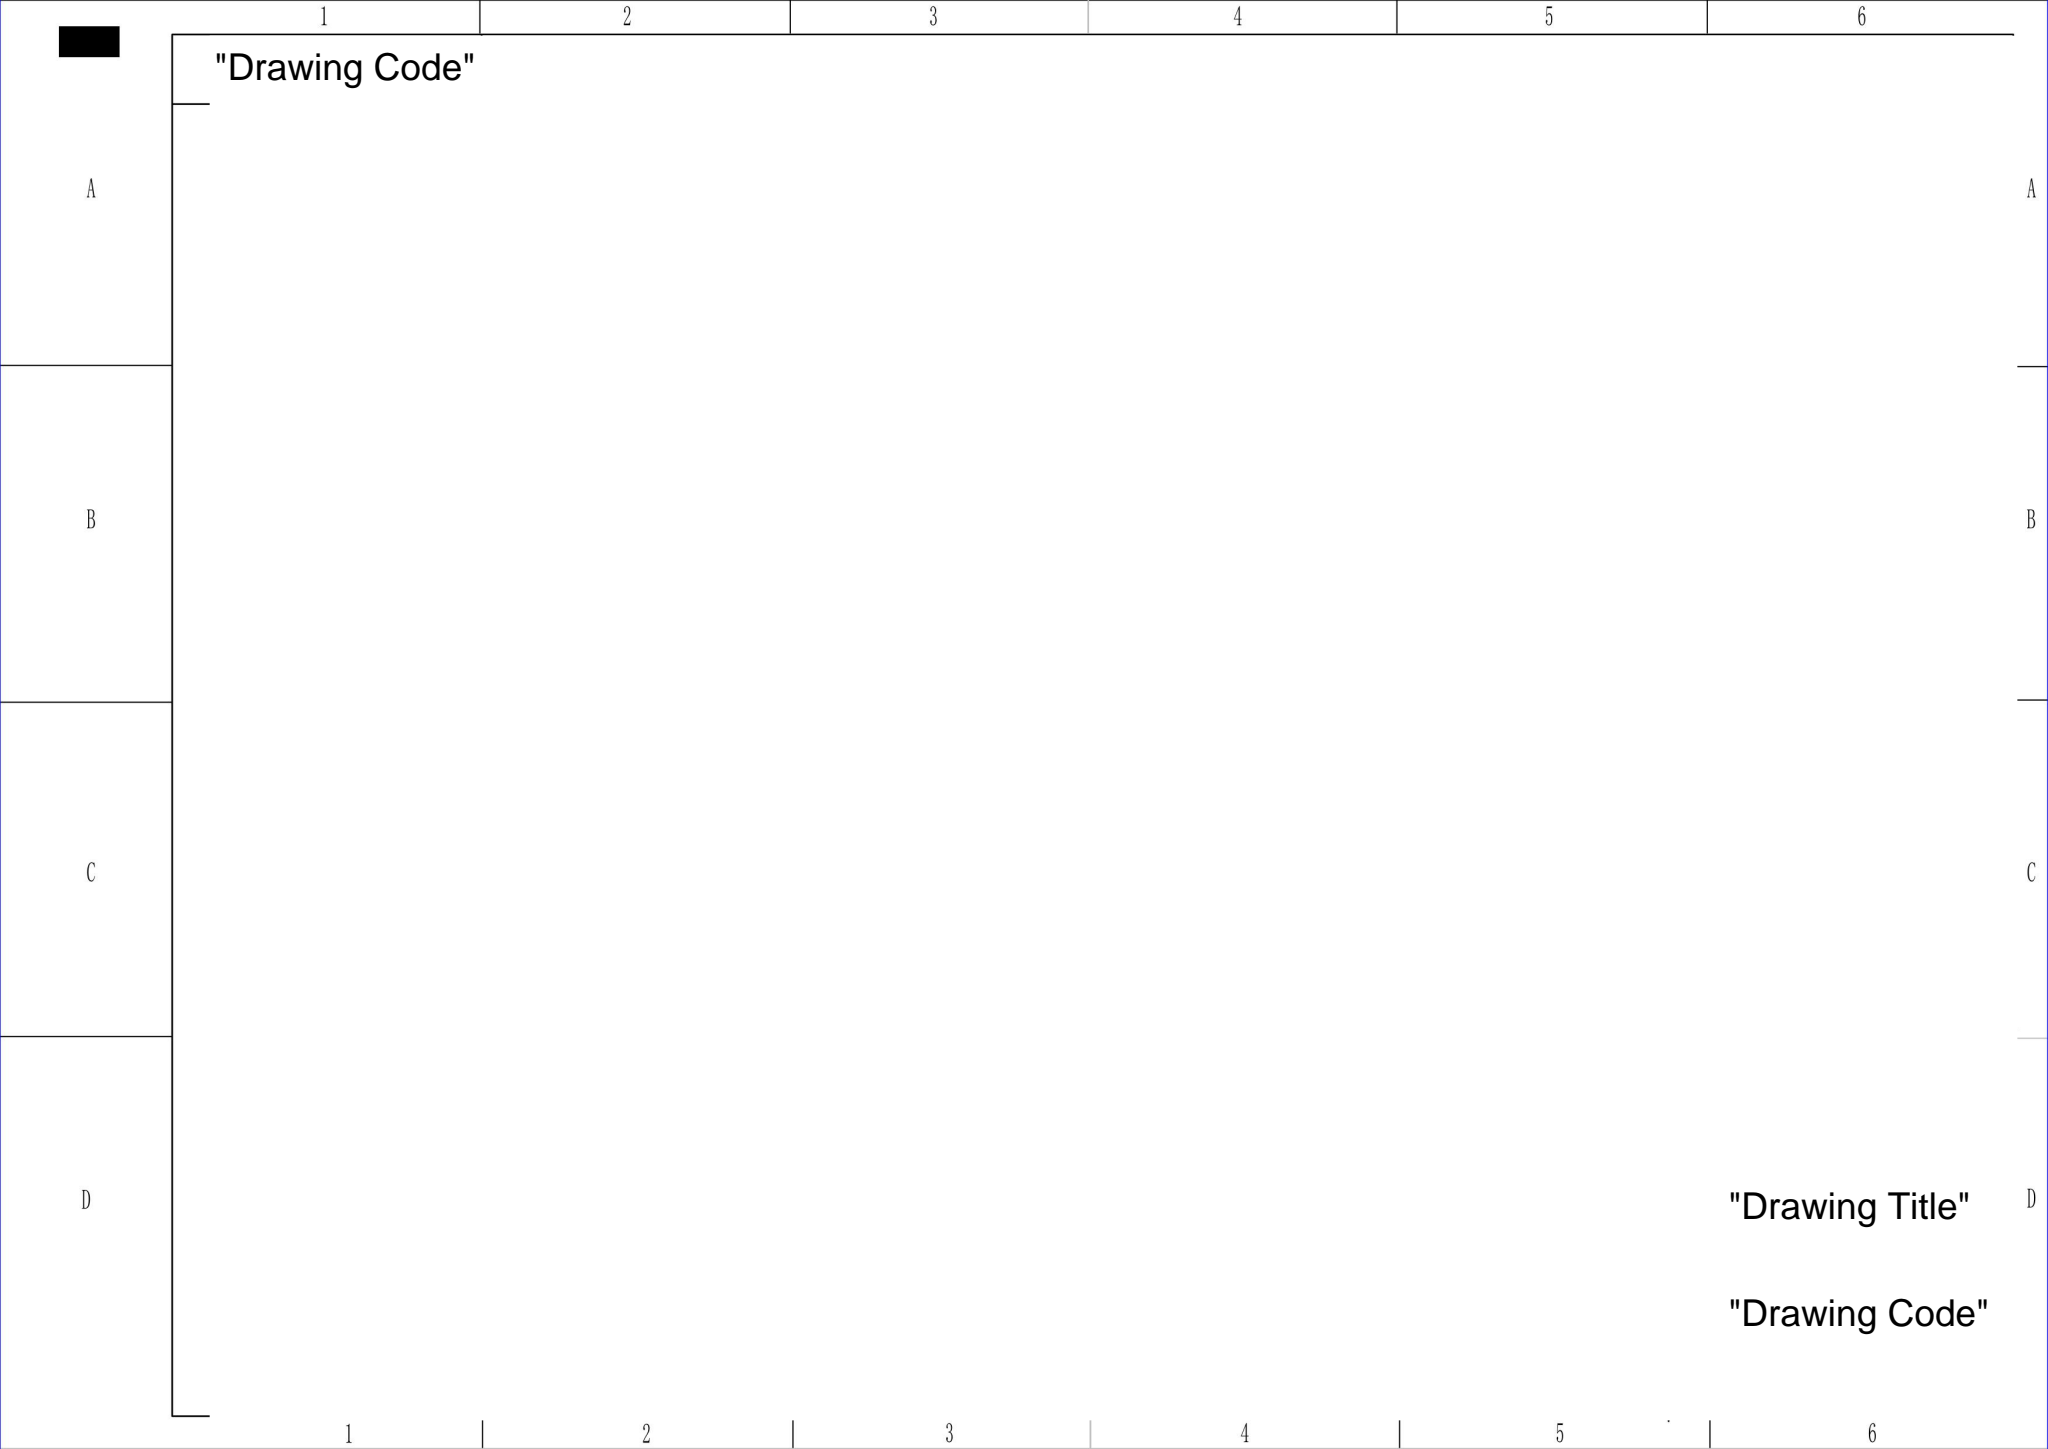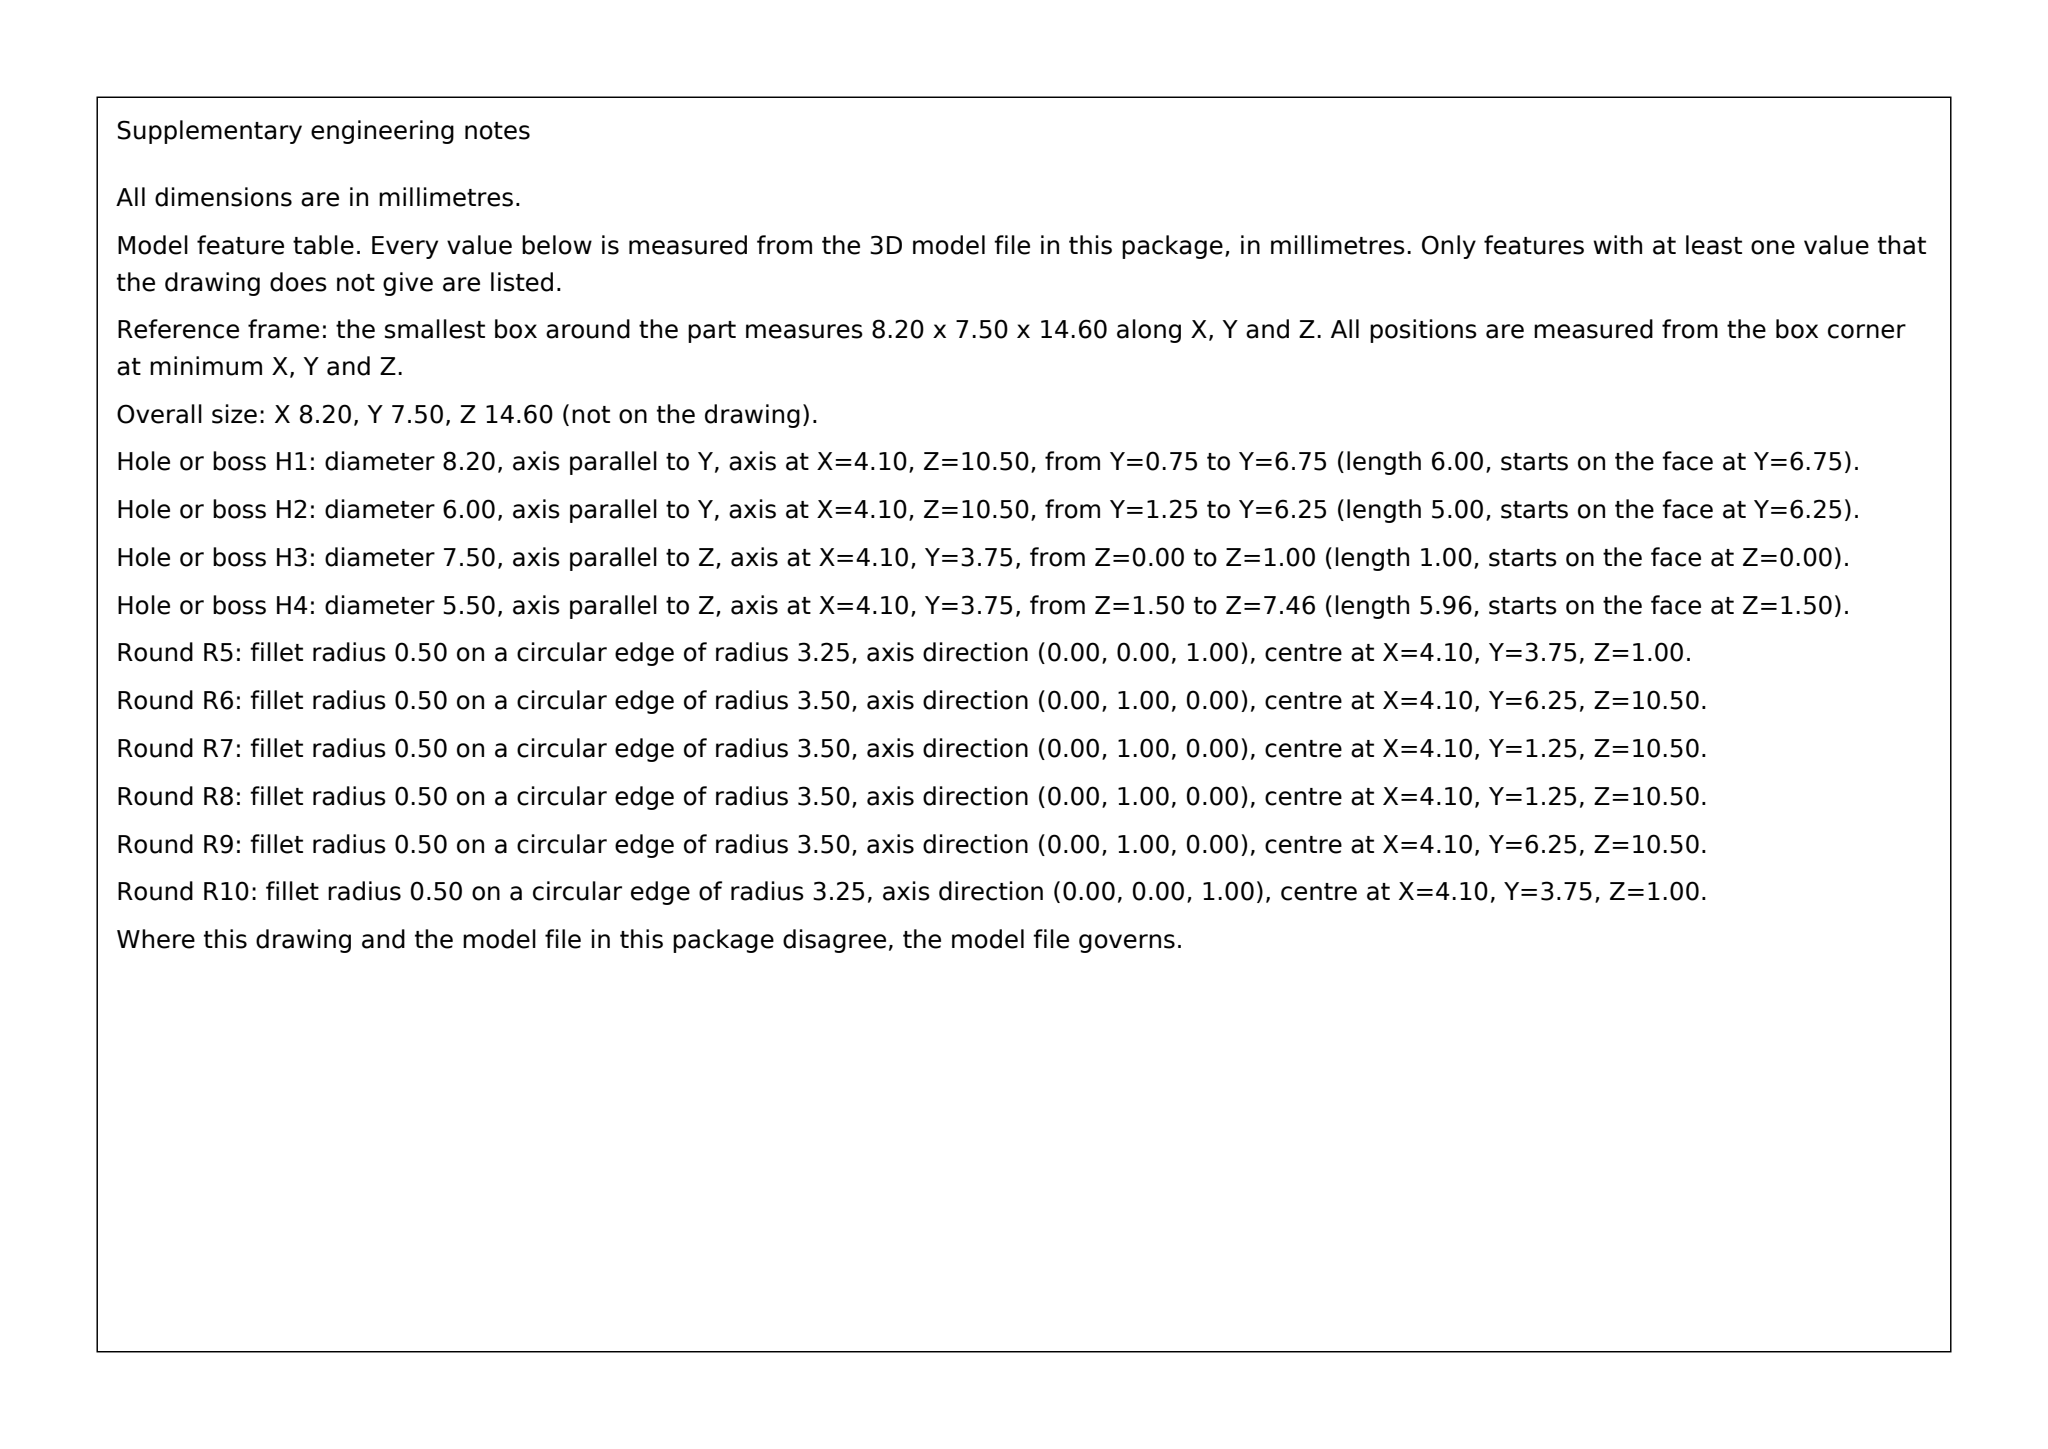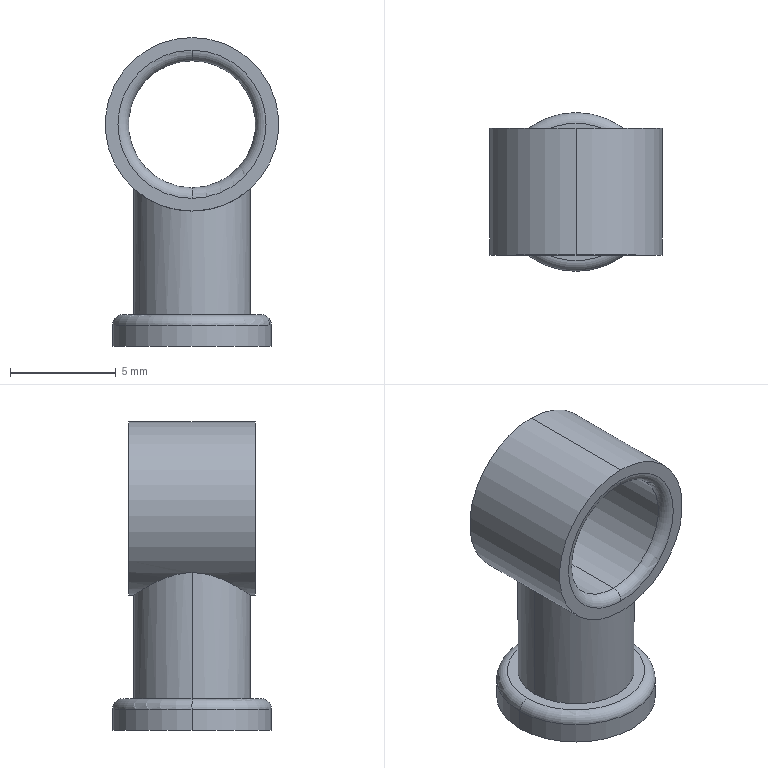Part | SolidWorks | mm | 1 solid | 18 faces | box 8.2 x 7.5 x 14.6 mm | volume 332 mm3 | cylinder 8 | torus 6 | plane 4 | commonest cylinder face diameters 6 x2 8.2 x2 7.5 x2 5.5 x2
STEP:
#1=CARTESIAN_POINT('',(-3.75,0.,1.));
#2=VERTEX_POINT('',#1);
#3=CARTESIAN_POINT('',(3.75,0.,1.));
#4=VERTEX_POINT('',#3);
#5=CARTESIAN_POINT('',(0.,0.,1.));
#6=DIRECTION('',(0.,0.,-1.));
#7=DIRECTION('',(1.,0.,0.));
#8=AXIS2_PLACEMENT_3D('',#5,#6,#7);
#9=CIRCLE('',#8,3.75);
#10=EDGE_CURVE('',#2,#4,#9,.T.);
#11=ORIENTED_EDGE('',*,*,#10,.F.);
#12=CARTESIAN_POINT('',(-3.25,0.,1.5));
#13=VERTEX_POINT('',#12);
#14=CARTESIAN_POINT('',(-3.25,0.,1.));
#15=DIRECTION('',(0.,1.,0.));
#16=DIRECTION('',(-1.,0.,0.));
#17=AXIS2_PLACEMENT_3D('',#14,#15,#16);
#18=CIRCLE('',#17,0.5);
#19=EDGE_CURVE('',#2,#13,#18,.T.);
#20=ORIENTED_EDGE('',*,*,#19,.T.);
#21=CARTESIAN_POINT('',(3.25,0.,1.5));
#22=VERTEX_POINT('',#21);
#23=CARTESIAN_POINT('',(0.,0.,1.5));
#24=DIRECTION('',(0.,0.,1.));
#25=DIRECTION('',(1.,0.,0.));
#26=AXIS2_PLACEMENT_3D('',#23,#24,#25);
#27=CIRCLE('',#26,3.25);
#28=EDGE_CURVE('',#22,#13,#27,.T.);
#29=ORIENTED_EDGE('',*,*,#28,.F.);
#30=CARTESIAN_POINT('',(3.25,0.,1.));
#31=DIRECTION('',(0.,-1.,0.));
#32=DIRECTION('',(0.,0.,-1.));
#33=AXIS2_PLACEMENT_3D('',#30,#31,#32);
#34=CIRCLE('',#33,0.5);
#35=EDGE_CURVE('',#4,#22,#34,.T.);
#36=ORIENTED_EDGE('',*,*,#35,.F.);
#37=EDGE_LOOP('',(#11,#20,#29,#36));
#38=FACE_OUTER_BOUND('',#37,.T.);
#39=CARTESIAN_POINT('',(0.,0.,1.));
#40=DIRECTION('',(0.,0.,1.));
#41=DIRECTION('',(1.,0.,0.));
#42=AXIS2_PLACEMENT_3D('',#39,#40,#41);
#43=TOROIDAL_SURFACE('',#42,3.25,0.5);
#44=ADVANCED_FACE('',(#38),#43,.T.);
#45=CARTESIAN_POINT('',(0.,3.,7.));
#46=VERTEX_POINT('',#45);
#47=CARTESIAN_POINT('',(0.,3.,14.));
#48=VERTEX_POINT('',#47);
#49=CARTESIAN_POINT('',(0.,3.,10.5));
#50=DIRECTION('',(0.,-1.,0.));
#51=DIRECTION('',(0.,0.,1.));
#52=AXIS2_PLACEMENT_3D('',#49,#50,#51);
#53=CIRCLE('',#52,3.5);
#54=EDGE_CURVE('',#46,#48,#53,.T.);
#55=ORIENTED_EDGE('',*,*,#54,.F.);
#56=CARTESIAN_POINT('',(0.,2.5,7.5));
#57=VERTEX_POINT('',#56);
#58=CARTESIAN_POINT('',(0.,2.5,7.));
#59=DIRECTION('',(1.,0.,0.));
#60=DIRECTION('',(0.,0.,-1.));
#61=AXIS2_PLACEMENT_3D('',#58,#59,#60);
#62=CIRCLE('',#61,0.5);
#63=EDGE_CURVE('',#46,#57,#62,.T.);
#64=ORIENTED_EDGE('',*,*,#63,.T.);
#65=CARTESIAN_POINT('',(0.,2.5,13.5));
#66=VERTEX_POINT('',#65);
#67=CARTESIAN_POINT('',(0.,2.5,10.5));
#68=DIRECTION('',(0.,1.,0.));
#69=DIRECTION('',(0.,0.,1.));
#70=AXIS2_PLACEMENT_3D('',#67,#68,#69);
#71=CIRCLE('',#70,3.);
#72=EDGE_CURVE('',#66,#57,#71,.T.);
#73=ORIENTED_EDGE('',*,*,#72,.F.);
#74=CARTESIAN_POINT('',(0.,2.5,14.));
#75=DIRECTION('',(-1.,0.,0.));
#76=DIRECTION('',(0.,0.,1.));
#77=AXIS2_PLACEMENT_3D('',#74,#75,#76);
#78=CIRCLE('',#77,0.5);
#79=EDGE_CURVE('',#48,#66,#78,.T.);
#80=ORIENTED_EDGE('',*,*,#79,.F.);
#81=EDGE_LOOP('',(#55,#64,#73,#80));
#82=FACE_OUTER_BOUND('',#81,.T.);
#83=CARTESIAN_POINT('',(0.,2.5,10.5));
#84=DIRECTION('',(0.,1.,0.));
#85=DIRECTION('',(0.,0.,1.));
#86=AXIS2_PLACEMENT_3D('',#83,#84,#85);
#87=TOROIDAL_SURFACE('',#86,3.5,0.5);
#88=ADVANCED_FACE('',(#82),#87,.T.);
#89=CARTESIAN_POINT('',(0.,-2.5,7.5));
#90=VERTEX_POINT('',#89);
#91=CARTESIAN_POINT('',(0.,-2.5,13.5));
#92=VERTEX_POINT('',#91);
#93=CARTESIAN_POINT('',(0.,-2.5,10.5));
#94=DIRECTION('',(0.,-1.,0.));
#95=DIRECTION('',(0.,0.,1.));
#96=AXIS2_PLACEMENT_3D('',#93,#94,#95);
#97=CIRCLE('',#96,3.);
#98=EDGE_CURVE('',#90,#92,#97,.T.);
#99=ORIENTED_EDGE('',*,*,#98,.F.);
#100=CARTESIAN_POINT('',(0.,-3.,7.));
#101=VERTEX_POINT('',#100);
#102=CARTESIAN_POINT('',(0.,-2.5,7.));
#103=DIRECTION('',(1.,0.,0.));
#104=DIRECTION('',(0.,0.,-1.));
#105=AXIS2_PLACEMENT_3D('',#102,#103,#104);
#106=CIRCLE('',#105,0.5);
#107=EDGE_CURVE('',#90,#101,#106,.T.);
#108=ORIENTED_EDGE('',*,*,#107,.T.);
#109=CARTESIAN_POINT('',(0.,-3.,14.));
#110=VERTEX_POINT('',#109);
#111=CARTESIAN_POINT('',(0.,-3.,10.5));
#112=DIRECTION('',(0.,1.,0.));
#113=DIRECTION('',(0.,0.,1.));
#114=AXIS2_PLACEMENT_3D('',#111,#112,#113);
#115=CIRCLE('',#114,3.5);
#116=EDGE_CURVE('',#110,#101,#115,.T.);
#117=ORIENTED_EDGE('',*,*,#116,.F.);
#118=CARTESIAN_POINT('',(0.,-2.5,14.));
#119=DIRECTION('',(-1.,0.,0.));
#120=DIRECTION('',(0.,0.,1.));
#121=AXIS2_PLACEMENT_3D('',#118,#119,#120);
#122=CIRCLE('',#121,0.5);
#123=EDGE_CURVE('',#92,#110,#122,.T.);
#124=ORIENTED_EDGE('',*,*,#123,.F.);
#125=EDGE_LOOP('',(#99,#108,#117,#124));
#126=FACE_OUTER_BOUND('',#125,.T.);
#127=CARTESIAN_POINT('',(0.,-2.5,10.5));
#128=DIRECTION('',(0.,1.,0.));
#129=DIRECTION('',(0.,0.,1.));
#130=AXIS2_PLACEMENT_3D('',#127,#128,#129);
#131=TOROIDAL_SURFACE('',#130,3.5,0.5);
#132=ADVANCED_FACE('',(#126),#131,.T.);
#133=CARTESIAN_POINT('',(0.,2.5,10.5));
#134=DIRECTION('',(0.,1.,0.));
#135=DIRECTION('',(0.,0.,1.));
#136=AXIS2_PLACEMENT_3D('',#133,#134,#135);
#137=CIRCLE('',#136,3.);
#138=EDGE_CURVE('',#57,#66,#137,.T.);
#139=ORIENTED_EDGE('',*,*,#138,.T.);
#140=CARTESIAN_POINT('',(0.,3.,13.5));
#141=DIRECTION('',(0.,-1.,0.));
#142=VECTOR('',#141,1000.);
#143=LINE('',#140,#142);
#144=EDGE_CURVE('',#66,#92,#143,.T.);
#145=ORIENTED_EDGE('',*,*,#144,.T.);
#146=CARTESIAN_POINT('',(0.,-2.5,10.5));
#147=DIRECTION('',(0.,-1.,0.));
#148=DIRECTION('',(0.,0.,1.));
#149=AXIS2_PLACEMENT_3D('',#146,#147,#148);
#150=CIRCLE('',#149,3.);
#151=EDGE_CURVE('',#92,#90,#150,.T.);
#152=ORIENTED_EDGE('',*,*,#151,.T.);
#153=CARTESIAN_POINT('',(0.,3.,7.5));
#154=DIRECTION('',(0.,-1.,0.));
#155=VECTOR('',#154,1000.);
#156=LINE('',#153,#155);
#157=EDGE_CURVE('',#57,#90,#156,.T.);
#158=ORIENTED_EDGE('',*,*,#157,.F.);
#159=EDGE_LOOP('',(#139,#145,#152,#158));
#160=FACE_OUTER_BOUND('',#159,.T.);
#161=CARTESIAN_POINT('',(0.,3.,10.5));
#162=DIRECTION('',(0.,-1.,0.));
#163=DIRECTION('',(0.,0.,-1.));
#164=AXIS2_PLACEMENT_3D('',#161,#162,#163);
#165=CYLINDRICAL_SURFACE('',#164,3.);
#166=ADVANCED_FACE('',(#160),#165,.F.);
#167=CARTESIAN_POINT('',(0.,3.,14.6));
#168=VERTEX_POINT('',#167);
#169=CARTESIAN_POINT('',(0.,3.,6.4));
#170=VERTEX_POINT('',#169);
#171=CARTESIAN_POINT('',(0.,3.,10.5));
#172=DIRECTION('',(0.,1.,0.));
#173=DIRECTION('',(0.,0.,1.));
#174=AXIS2_PLACEMENT_3D('',#171,#172,#173);
#175=CIRCLE('',#174,4.1);
#176=EDGE_CURVE('',#168,#170,#175,.T.);
#177=ORIENTED_EDGE('',*,*,#176,.F.);
#178=CARTESIAN_POINT('',(0.,-3.,14.6));
#179=VERTEX_POINT('',#178);
#180=CARTESIAN_POINT('',(0.,3.,14.6));
#181=DIRECTION('',(0.,-1.,0.));
#182=VECTOR('',#181,1000.);
#183=LINE('',#180,#182);
#184=EDGE_CURVE('',#168,#179,#183,.T.);
#185=ORIENTED_EDGE('',*,*,#184,.T.);
#186=CARTESIAN_POINT('',(0.,-3.,6.4));
#187=VERTEX_POINT('',#186);
#188=CARTESIAN_POINT('',(0.,-3.,10.5));
#189=DIRECTION('',(0.,1.,0.));
#190=DIRECTION('',(0.,0.,1.));
#191=AXIS2_PLACEMENT_3D('',#188,#189,#190);
#192=CIRCLE('',#191,4.1);
#193=EDGE_CURVE('',#179,#187,#192,.T.);
#194=ORIENTED_EDGE('',*,*,#193,.T.);
#195=CARTESIAN_POINT('',(0.,-2.75,6.4));
#196=VERTEX_POINT('',#195);
#197=CARTESIAN_POINT('',(0.,3.,6.4));
#198=DIRECTION('',(0.,-1.,0.));
#199=VECTOR('',#198,1000.);
#200=LINE('',#197,#199);
#201=EDGE_CURVE('',#196,#187,#200,.T.);
#202=ORIENTED_EDGE('',*,*,#201,.F.);
#203=CARTESIAN_POINT('',(2.75,0.,7.459));
#204=VERTEX_POINT('',#203);
#205=CARTESIAN_POINT('',(0.,-2.75,6.4));
#206=CARTESIAN_POINT('',(0.1875,-2.75,6.4));
#207=CARTESIAN_POINT('',(0.3733,-2.731,6.413));
#208=CARTESIAN_POINT('',(0.734,-2.657,6.462));
#209=CARTESIAN_POINT('',(0.9116,-2.601,6.499));
#210=CARTESIAN_POINT('',(1.41,-2.389,6.635));
#211=CARTESIAN_POINT('',(1.706,-2.185,6.761));
#212=CARTESIAN_POINT('',(2.074,-1.815,6.96));
#213=CARTESIAN_POINT('',(2.185,-1.678,7.029));
#214=CARTESIAN_POINT('',(2.379,-1.39,7.159));
#215=CARTESIAN_POINT('',(2.463,-1.236,7.221));
#216=CARTESIAN_POINT('',(2.602,-0.9088,7.33));
#217=CARTESIAN_POINT('',(2.657,-0.7333,7.377));
#218=CARTESIAN_POINT('',(2.731,-0.3747,7.441));
#219=CARTESIAN_POINT('',(2.75,-0.1864,7.459));
#220=CARTESIAN_POINT('',(2.75,0.,7.459));
#221=B_SPLINE_CURVE_WITH_KNOTS('',3,(#205,#206,#207,#208,#209,#210,#211,#212,#213,#214,#215,#216,#217,#218,#219,#220),.UNSPECIFIED.,.F.,.F.,(4,2,2,2,2,2,2,4),(0.00445,0.005005,0.005559,0.006668,0.007223,0.007777,0.008332,0.008886),.UNSPECIFIED.);
#222=EDGE_CURVE('',#196,#204,#221,.T.);
#223=ORIENTED_EDGE('',*,*,#222,.T.);
#224=CARTESIAN_POINT('',(-0.,2.75,6.4));
#225=VERTEX_POINT('',#224);
#226=CARTESIAN_POINT('',(2.75,0.,7.459));
#227=CARTESIAN_POINT('',(2.75,0.1864,7.459));
#228=CARTESIAN_POINT('',(2.731,0.3704,7.442));
#229=CARTESIAN_POINT('',(2.657,0.7339,7.377));
#230=CARTESIAN_POINT('',(2.602,0.9064,7.331));
#231=CARTESIAN_POINT('',(2.463,1.236,7.221));
#232=CARTESIAN_POINT('',(2.378,1.392,7.158));
#233=CARTESIAN_POINT('',(2.184,1.68,7.028));
#234=CARTESIAN_POINT('',(2.074,1.814,6.961));
#235=CARTESIAN_POINT('',(1.704,2.187,6.76));
#236=CARTESIAN_POINT('',(1.414,2.387,6.636));
#237=CARTESIAN_POINT('',(0.9105,2.601,6.499));
#238=CARTESIAN_POINT('',(0.7363,2.656,6.463));
#239=CARTESIAN_POINT('',(0.3747,2.731,6.413));
#240=CARTESIAN_POINT('',(0.1857,2.75,6.4));
#241=CARTESIAN_POINT('',(-0.,2.75,6.4));
#242=B_SPLINE_CURVE_WITH_KNOTS('',3,(#226,#227,#228,#229,#230,#231,#232,#233,#234,#235,#236,#237,#238,#239,#240,#241),.UNSPECIFIED.,.F.,.F.,(4,2,2,2,2,2,2,4),(0.008886,0.009441,0.009995,0.01055,0.0111,0.01221,0.01277,0.01332),.UNSPECIFIED.);
#243=EDGE_CURVE('',#204,#225,#242,.T.);
#244=ORIENTED_EDGE('',*,*,#243,.T.);
#245=CARTESIAN_POINT('',(0.,3.,6.4));
#246=DIRECTION('',(0.,-1.,0.));
#247=VECTOR('',#246,1000.);
#248=LINE('',#245,#247);
#249=EDGE_CURVE('',#170,#225,#248,.T.);
#250=ORIENTED_EDGE('',*,*,#249,.F.);
#251=EDGE_LOOP('',(#177,#185,#194,#202,#223,#244,#250));
#252=FACE_OUTER_BOUND('',#251,.T.);
#253=CARTESIAN_POINT('',(0.,3.,10.5));
#254=DIRECTION('',(0.,-1.,0.));
#255=DIRECTION('',(0.,0.,-1.));
#256=AXIS2_PLACEMENT_3D('',#253,#254,#255);
#257=CYLINDRICAL_SURFACE('',#256,4.1);
#258=ADVANCED_FACE('',(#252),#257,.T.);
#259=ORIENTED_EDGE('',*,*,#10,.T.);
#260=CARTESIAN_POINT('',(3.75,0.,0.));
#261=VERTEX_POINT('',#260);
#262=CARTESIAN_POINT('',(3.75,0.,1.5));
#263=DIRECTION('',(0.,0.,-1.));
#264=VECTOR('',#263,1000.);
#265=LINE('',#262,#264);
#266=EDGE_CURVE('',#4,#261,#265,.T.);
#267=ORIENTED_EDGE('',*,*,#266,.T.);
#268=CARTESIAN_POINT('',(-3.75,0.,0.));
#269=VERTEX_POINT('',#268);
#270=CARTESIAN_POINT('',(0.,0.,0.));
#271=DIRECTION('',(0.,0.,1.));
#272=DIRECTION('',(1.,0.,0.));
#273=AXIS2_PLACEMENT_3D('',#270,#271,#272);
#274=CIRCLE('',#273,3.75);
#275=EDGE_CURVE('',#261,#269,#274,.T.);
#276=ORIENTED_EDGE('',*,*,#275,.T.);
#277=CARTESIAN_POINT('',(-3.75,0.,1.5));
#278=DIRECTION('',(0.,0.,-1.));
#279=VECTOR('',#278,1000.);
#280=LINE('',#277,#279);
#281=EDGE_CURVE('',#2,#269,#280,.T.);
#282=ORIENTED_EDGE('',*,*,#281,.F.);
#283=EDGE_LOOP('',(#259,#267,#276,#282));
#284=FACE_OUTER_BOUND('',#283,.T.);
#285=CARTESIAN_POINT('',(0.,0.,1.5));
#286=DIRECTION('',(0.,0.,-1.));
#287=DIRECTION('',(-1.,0.,0.));
#288=AXIS2_PLACEMENT_3D('',#285,#286,#287);
#289=CYLINDRICAL_SURFACE('',#288,3.75);
#290=ADVANCED_FACE('',(#284),#289,.T.);
#291=ORIENTED_EDGE('',*,*,#243,.F.);
#292=CARTESIAN_POINT('',(2.75,0.,1.5));
#293=VERTEX_POINT('',#292);
#294=CARTESIAN_POINT('',(2.75,0.,7.5));
#295=DIRECTION('',(0.,0.,-1.));
#296=VECTOR('',#295,1000.);
#297=LINE('',#294,#296);
#298=EDGE_CURVE('',#204,#293,#297,.T.);
#299=ORIENTED_EDGE('',*,*,#298,.T.);
#300=CARTESIAN_POINT('',(-2.75,0.,1.5));
#301=VERTEX_POINT('',#300);
#302=CARTESIAN_POINT('',(0.,0.,1.5));
#303=DIRECTION('',(0.,0.,1.));
#304=DIRECTION('',(1.,0.,0.));
#305=AXIS2_PLACEMENT_3D('',#302,#303,#304);
#306=CIRCLE('',#305,2.75);
#307=EDGE_CURVE('',#293,#301,#306,.T.);
#308=ORIENTED_EDGE('',*,*,#307,.T.);
#309=CARTESIAN_POINT('',(-2.75,-0.,7.459));
#310=VERTEX_POINT('',#309);
#311=CARTESIAN_POINT('',(-2.75,0.,7.5));
#312=DIRECTION('',(0.,0.,-1.));
#313=VECTOR('',#312,1000.);
#314=LINE('',#311,#313);
#315=EDGE_CURVE('',#310,#301,#314,.T.);
#316=ORIENTED_EDGE('',*,*,#315,.F.);
#317=CARTESIAN_POINT('',(-0.,2.75,6.4));
#318=CARTESIAN_POINT('',(-0.1854,2.75,6.4));
#319=CARTESIAN_POINT('',(-0.3712,2.731,6.413));
#320=CARTESIAN_POINT('',(-0.7352,2.656,6.462));
#321=CARTESIAN_POINT('',(-0.9091,2.602,6.498));
#322=CARTESIAN_POINT('',(-1.242,2.46,6.589));
#323=CARTESIAN_POINT('',(-1.401,2.373,6.643));
#324=CARTESIAN_POINT('',(-1.692,2.175,6.762));
#325=CARTESIAN_POINT('',(-1.828,2.062,6.827));
#326=CARTESIAN_POINT('',(-2.074,1.815,6.96));
#327=CARTESIAN_POINT('',(-2.183,1.681,7.028));
#328=CARTESIAN_POINT('',(-2.378,1.392,7.158));
#329=CARTESIAN_POINT('',(-2.463,1.236,7.221));
#330=CARTESIAN_POINT('',(-2.602,0.9082,7.33));
#331=CARTESIAN_POINT('',(-2.656,0.7366,7.376));
#332=CARTESIAN_POINT('',(-2.731,0.3734,7.441));
#333=CARTESIAN_POINT('',(-2.75,0.1879,7.459));
#334=CARTESIAN_POINT('',(-2.75,-0.,7.459));
#335=B_SPLINE_CURVE_WITH_KNOTS('',3,(#317,#318,#319,#320,#321,#322,#323,#324,#325,#326,#327,#328,#329,#330,#331,#332,#333,#334),.UNSPECIFIED.,.F.,.F.,(4,2,2,2,2,2,2,2,4),(0.01332,0.01388,0.01443,0.01498,0.01554,0.01609,0.01664,0.0172,0.01775),.UNSPECIFIED.);
#336=EDGE_CURVE('',#225,#310,#335,.T.);
#337=ORIENTED_EDGE('',*,*,#336,.F.);
#338=EDGE_LOOP('',(#291,#299,#308,#316,#337));
#339=FACE_OUTER_BOUND('',#338,.T.);
#340=CARTESIAN_POINT('',(0.,0.,7.5));
#341=DIRECTION('',(0.,0.,-1.));
#342=DIRECTION('',(-1.,0.,0.));
#343=AXIS2_PLACEMENT_3D('',#340,#341,#342);
#344=CYLINDRICAL_SURFACE('',#343,2.75);
#345=ADVANCED_FACE('',(#339),#344,.T.);
#346=ORIENTED_EDGE('',*,*,#298,.F.);
#347=ORIENTED_EDGE('',*,*,#222,.F.);
#348=CARTESIAN_POINT('',(-2.75,-0.,7.459));
#349=CARTESIAN_POINT('',(-2.75,-0.1889,7.459));
#350=CARTESIAN_POINT('',(-2.731,-0.3727,7.441));
#351=CARTESIAN_POINT('',(-2.657,-0.7316,7.377));
#352=CARTESIAN_POINT('',(-2.602,-0.9075,7.33));
#353=CARTESIAN_POINT('',(-2.463,-1.236,7.221));
#354=CARTESIAN_POINT('',(-2.378,-1.391,7.158));
#355=CARTESIAN_POINT('',(-2.182,-1.683,7.027));
#356=CARTESIAN_POINT('',(-2.072,-1.817,6.959));
#357=CARTESIAN_POINT('',(-1.826,-2.064,6.826));
#358=CARTESIAN_POINT('',(-1.689,-2.177,6.761));
#359=CARTESIAN_POINT('',(-1.398,-2.375,6.642));
#360=CARTESIAN_POINT('',(-1.243,-2.46,6.589));
#361=CARTESIAN_POINT('',(-0.9103,-2.601,6.499));
#362=CARTESIAN_POINT('',(-0.732,-2.657,6.462));
#363=CARTESIAN_POINT('',(-0.372,-2.731,6.413));
#364=CARTESIAN_POINT('',(-0.1881,-2.75,6.4));
#365=CARTESIAN_POINT('',(0.,-2.75,6.4));
#366=B_SPLINE_CURVE_WITH_KNOTS('',3,(#348,#349,#350,#351,#352,#353,#354,#355,#356,#357,#358,#359,#360,#361,#362,#363,#364,#365),.UNSPECIFIED.,.F.,.F.,(4,2,2,2,2,2,2,2,4),(0.,0.0005563,0.001113,0.001669,0.002225,0.002782,0.003338,0.003894,0.00445),.UNSPECIFIED.);
#367=EDGE_CURVE('',#310,#196,#366,.T.);
#368=ORIENTED_EDGE('',*,*,#367,.F.);
#369=ORIENTED_EDGE('',*,*,#315,.T.);
#370=CARTESIAN_POINT('',(0.,0.,1.5));
#371=DIRECTION('',(0.,0.,1.));
#372=DIRECTION('',(1.,0.,0.));
#373=AXIS2_PLACEMENT_3D('',#370,#371,#372);
#374=CIRCLE('',#373,2.75);
#375=EDGE_CURVE('',#301,#293,#374,.T.);
#376=ORIENTED_EDGE('',*,*,#375,.T.);
#377=EDGE_LOOP('',(#346,#347,#368,#369,#376));
#378=FACE_OUTER_BOUND('',#377,.T.);
#379=CARTESIAN_POINT('',(0.,0.,7.5));
#380=DIRECTION('',(0.,0.,-1.));
#381=DIRECTION('',(-1.,0.,0.));
#382=AXIS2_PLACEMENT_3D('',#379,#380,#381);
#383=CYLINDRICAL_SURFACE('',#382,2.75);
#384=ADVANCED_FACE('',(#378),#383,.T.);
#385=ORIENTED_EDGE('',*,*,#266,.F.);
#386=CARTESIAN_POINT('',(0.,0.,1.));
#387=DIRECTION('',(0.,0.,-1.));
#388=DIRECTION('',(1.,0.,0.));
#389=AXIS2_PLACEMENT_3D('',#386,#387,#388);
#390=CIRCLE('',#389,3.75);
#391=EDGE_CURVE('',#4,#2,#390,.T.);
#392=ORIENTED_EDGE('',*,*,#391,.T.);
#393=ORIENTED_EDGE('',*,*,#281,.T.);
#394=CARTESIAN_POINT('',(0.,0.,0.));
#395=DIRECTION('',(0.,0.,1.));
#396=DIRECTION('',(1.,0.,0.));
#397=AXIS2_PLACEMENT_3D('',#394,#395,#396);
#398=CIRCLE('',#397,3.75);
#399=EDGE_CURVE('',#269,#261,#398,.T.);
#400=ORIENTED_EDGE('',*,*,#399,.T.);
#401=EDGE_LOOP('',(#385,#392,#393,#400));
#402=FACE_OUTER_BOUND('',#401,.T.);
#403=CARTESIAN_POINT('',(0.,0.,1.5));
#404=DIRECTION('',(0.,0.,-1.));
#405=DIRECTION('',(-1.,0.,0.));
#406=AXIS2_PLACEMENT_3D('',#403,#404,#405);
#407=CYLINDRICAL_SURFACE('',#406,3.75);
#408=ADVANCED_FACE('',(#402),#407,.T.);
#409=ORIENTED_EDGE('',*,*,#28,.T.);
#410=CARTESIAN_POINT('',(0.,0.,1.5));
#411=DIRECTION('',(0.,0.,1.));
#412=DIRECTION('',(1.,0.,0.));
#413=AXIS2_PLACEMENT_3D('',#410,#411,#412);
#414=CIRCLE('',#413,3.25);
#415=EDGE_CURVE('',#13,#22,#414,.T.);
#416=ORIENTED_EDGE('',*,*,#415,.T.);
#417=EDGE_LOOP('',(#409,#416));
#418=FACE_OUTER_BOUND('',#417,.T.);
#419=ORIENTED_EDGE('',*,*,#375,.F.);
#420=ORIENTED_EDGE('',*,*,#307,.F.);
#421=EDGE_LOOP('',(#419,#420));
#422=FACE_BOUND('',#421,.T.);
#423=CARTESIAN_POINT('',(0.,0.,1.5));
#424=DIRECTION('',(0.,0.,1.));
#425=DIRECTION('',(1.,0.,0.));
#426=AXIS2_PLACEMENT_3D('',#423,#424,#425);
#427=PLANE('',#426);
#428=ADVANCED_FACE('',(#418,#422),#427,.T.);
#429=ORIENTED_EDGE('',*,*,#399,.F.);
#430=ORIENTED_EDGE('',*,*,#275,.F.);
#431=EDGE_LOOP('',(#429,#430));
#432=FACE_OUTER_BOUND('',#431,.T.);
#433=CARTESIAN_POINT('',(0.,0.,0.));
#434=DIRECTION('',(0.,0.,1.));
#435=DIRECTION('',(1.,0.,0.));
#436=AXIS2_PLACEMENT_3D('',#433,#434,#435);
#437=PLANE('',#436);
#438=ADVANCED_FACE('',(#432),#437,.F.);
#439=ORIENTED_EDGE('',*,*,#184,.F.);
#440=CARTESIAN_POINT('',(0.,3.,10.5));
#441=DIRECTION('',(0.,1.,0.));
#442=DIRECTION('',(0.,0.,1.));
#443=AXIS2_PLACEMENT_3D('',#440,#441,#442);
#444=CIRCLE('',#443,4.1);
#445=EDGE_CURVE('',#170,#168,#444,.T.);
#446=ORIENTED_EDGE('',*,*,#445,.F.);
#447=ORIENTED_EDGE('',*,*,#249,.T.);
#448=ORIENTED_EDGE('',*,*,#336,.T.);
#449=ORIENTED_EDGE('',*,*,#367,.T.);
#450=ORIENTED_EDGE('',*,*,#201,.T.);
#451=CARTESIAN_POINT('',(0.,-3.,10.5));
#452=DIRECTION('',(0.,1.,0.));
#453=DIRECTION('',(0.,0.,1.));
#454=AXIS2_PLACEMENT_3D('',#451,#452,#453);
#455=CIRCLE('',#454,4.1);
#456=EDGE_CURVE('',#187,#179,#455,.T.);
#457=ORIENTED_EDGE('',*,*,#456,.T.);
#458=EDGE_LOOP('',(#439,#446,#447,#448,#449,#450,#457));
#459=FACE_OUTER_BOUND('',#458,.T.);
#460=CARTESIAN_POINT('',(0.,3.,10.5));
#461=DIRECTION('',(0.,-1.,0.));
#462=DIRECTION('',(0.,0.,-1.));
#463=AXIS2_PLACEMENT_3D('',#460,#461,#462);
#464=CYLINDRICAL_SURFACE('',#463,4.1);
#465=ADVANCED_FACE('',(#459),#464,.T.);
#466=CARTESIAN_POINT('',(0.,3.,10.5));
#467=DIRECTION('',(0.,-1.,0.));
#468=DIRECTION('',(0.,0.,1.));
#469=AXIS2_PLACEMENT_3D('',#466,#467,#468);
#470=CIRCLE('',#469,3.5);
#471=EDGE_CURVE('',#48,#46,#470,.T.);
#472=ORIENTED_EDGE('',*,*,#471,.T.);
#473=ORIENTED_EDGE('',*,*,#54,.T.);
#474=EDGE_LOOP('',(#472,#473));
#475=FACE_BOUND('',#474,.T.);
#476=ORIENTED_EDGE('',*,*,#445,.T.);
#477=ORIENTED_EDGE('',*,*,#176,.T.);
#478=EDGE_LOOP('',(#476,#477));
#479=FACE_OUTER_BOUND('',#478,.T.);
#480=CARTESIAN_POINT('',(0.,3.,10.5));
#481=DIRECTION('',(0.,1.,0.));
#482=DIRECTION('',(0.,0.,1.));
#483=AXIS2_PLACEMENT_3D('',#480,#481,#482);
#484=PLANE('',#483);
#485=ADVANCED_FACE('',(#475,#479),#484,.T.);
#486=ORIENTED_EDGE('',*,*,#116,.T.);
#487=CARTESIAN_POINT('',(0.,-3.,10.5));
#488=DIRECTION('',(0.,1.,0.));
#489=DIRECTION('',(0.,0.,1.));
#490=AXIS2_PLACEMENT_3D('',#487,#488,#489);
#491=CIRCLE('',#490,3.5);
#492=EDGE_CURVE('',#101,#110,#491,.T.);
#493=ORIENTED_EDGE('',*,*,#492,.T.);
#494=EDGE_LOOP('',(#486,#493));
#495=FACE_BOUND('',#494,.T.);
#496=ORIENTED_EDGE('',*,*,#456,.F.);
#497=ORIENTED_EDGE('',*,*,#193,.F.);
#498=EDGE_LOOP('',(#496,#497));
#499=FACE_OUTER_BOUND('',#498,.T.);
#500=CARTESIAN_POINT('',(0.,-3.,10.5));
#501=DIRECTION('',(0.,1.,0.));
#502=DIRECTION('',(0.,0.,1.));
#503=AXIS2_PLACEMENT_3D('',#500,#501,#502);
#504=PLANE('',#503);
#505=ADVANCED_FACE('',(#495,#499),#504,.F.);
#506=ORIENTED_EDGE('',*,*,#144,.F.);
#507=ORIENTED_EDGE('',*,*,#72,.T.);
#508=ORIENTED_EDGE('',*,*,#157,.T.);
#509=ORIENTED_EDGE('',*,*,#98,.T.);
#510=EDGE_LOOP('',(#506,#507,#508,#509));
#511=FACE_OUTER_BOUND('',#510,.T.);
#512=CARTESIAN_POINT('',(0.,3.,10.5));
#513=DIRECTION('',(0.,-1.,0.));
#514=DIRECTION('',(0.,0.,-1.));
#515=AXIS2_PLACEMENT_3D('',#512,#513,#514);
#516=CYLINDRICAL_SURFACE('',#515,3.);
#517=ADVANCED_FACE('',(#511),#516,.F.);
#518=ORIENTED_EDGE('',*,*,#107,.F.);
#519=ORIENTED_EDGE('',*,*,#151,.F.);
#520=ORIENTED_EDGE('',*,*,#123,.T.);
#521=ORIENTED_EDGE('',*,*,#492,.F.);
#522=EDGE_LOOP('',(#518,#519,#520,#521));
#523=FACE_OUTER_BOUND('',#522,.T.);
#524=CARTESIAN_POINT('',(0.,-2.5,10.5));
#525=DIRECTION('',(0.,1.,0.));
#526=DIRECTION('',(0.,0.,1.));
#527=AXIS2_PLACEMENT_3D('',#524,#525,#526);
#528=TOROIDAL_SURFACE('',#527,3.5,0.5);
#529=ADVANCED_FACE('',(#523),#528,.T.);
#530=ORIENTED_EDGE('',*,*,#63,.F.);
#531=ORIENTED_EDGE('',*,*,#471,.F.);
#532=ORIENTED_EDGE('',*,*,#79,.T.);
#533=ORIENTED_EDGE('',*,*,#138,.F.);
#534=EDGE_LOOP('',(#530,#531,#532,#533));
#535=FACE_OUTER_BOUND('',#534,.T.);
#536=CARTESIAN_POINT('',(0.,2.5,10.5));
#537=DIRECTION('',(0.,1.,0.));
#538=DIRECTION('',(0.,0.,1.));
#539=AXIS2_PLACEMENT_3D('',#536,#537,#538);
#540=TOROIDAL_SURFACE('',#539,3.5,0.5);
#541=ADVANCED_FACE('',(#535),#540,.T.);
#542=ORIENTED_EDGE('',*,*,#19,.F.);
#543=ORIENTED_EDGE('',*,*,#391,.F.);
#544=ORIENTED_EDGE('',*,*,#35,.T.);
#545=ORIENTED_EDGE('',*,*,#415,.F.);
#546=EDGE_LOOP('',(#542,#543,#544,#545));
#547=FACE_OUTER_BOUND('',#546,.T.);
#548=CARTESIAN_POINT('',(0.,0.,1.));
#549=DIRECTION('',(0.,0.,1.));
#550=DIRECTION('',(1.,0.,0.));
#551=AXIS2_PLACEMENT_3D('',#548,#549,#550);
#552=TOROIDAL_SURFACE('',#551,3.25,0.5);
#553=ADVANCED_FACE('',(#547),#552,.T.);
#554=CLOSED_SHELL('',(#44,#88,#132,#166,#258,#290,#345,#384,#408,#428,#438,#465,#485,#505,#517,#529,#541,#553));
#555=MANIFOLD_SOLID_BREP('',#554);
#556=CARTESIAN_POINT('',(0.,0.,0.));
#557=DIRECTION('',(0.,0.,1.));
#558=DIRECTION('',(1.,0.,0.));
#559=AXIS2_PLACEMENT_3D('',#556,#557,#558);
#560=(LENGTH_UNIT()NAMED_UNIT(*)SI_UNIT(.MILLI.,.METRE.));
#561=UNCERTAINTY_MEASURE_WITH_UNIT(LENGTH_MEASURE(0.00001),#560,'','');
#562=(NAMED_UNIT(*)PLANE_ANGLE_UNIT()SI_UNIT($,.RADIAN.));
#563=(NAMED_UNIT(*)SI_UNIT($,.STERADIAN.)SOLID_ANGLE_UNIT());
#564=(GEOMETRIC_REPRESENTATION_CONTEXT(3)GLOBAL_UNCERTAINTY_ASSIGNED_CONTEXT((#561))GLOBAL_UNIT_ASSIGNED_CONTEXT((#560,#562,#563))REPRESENTATION_CONTEXT('',''));
#565=ADVANCED_BREP_SHAPE_REPRESENTATION('',(#555,#559),#564);